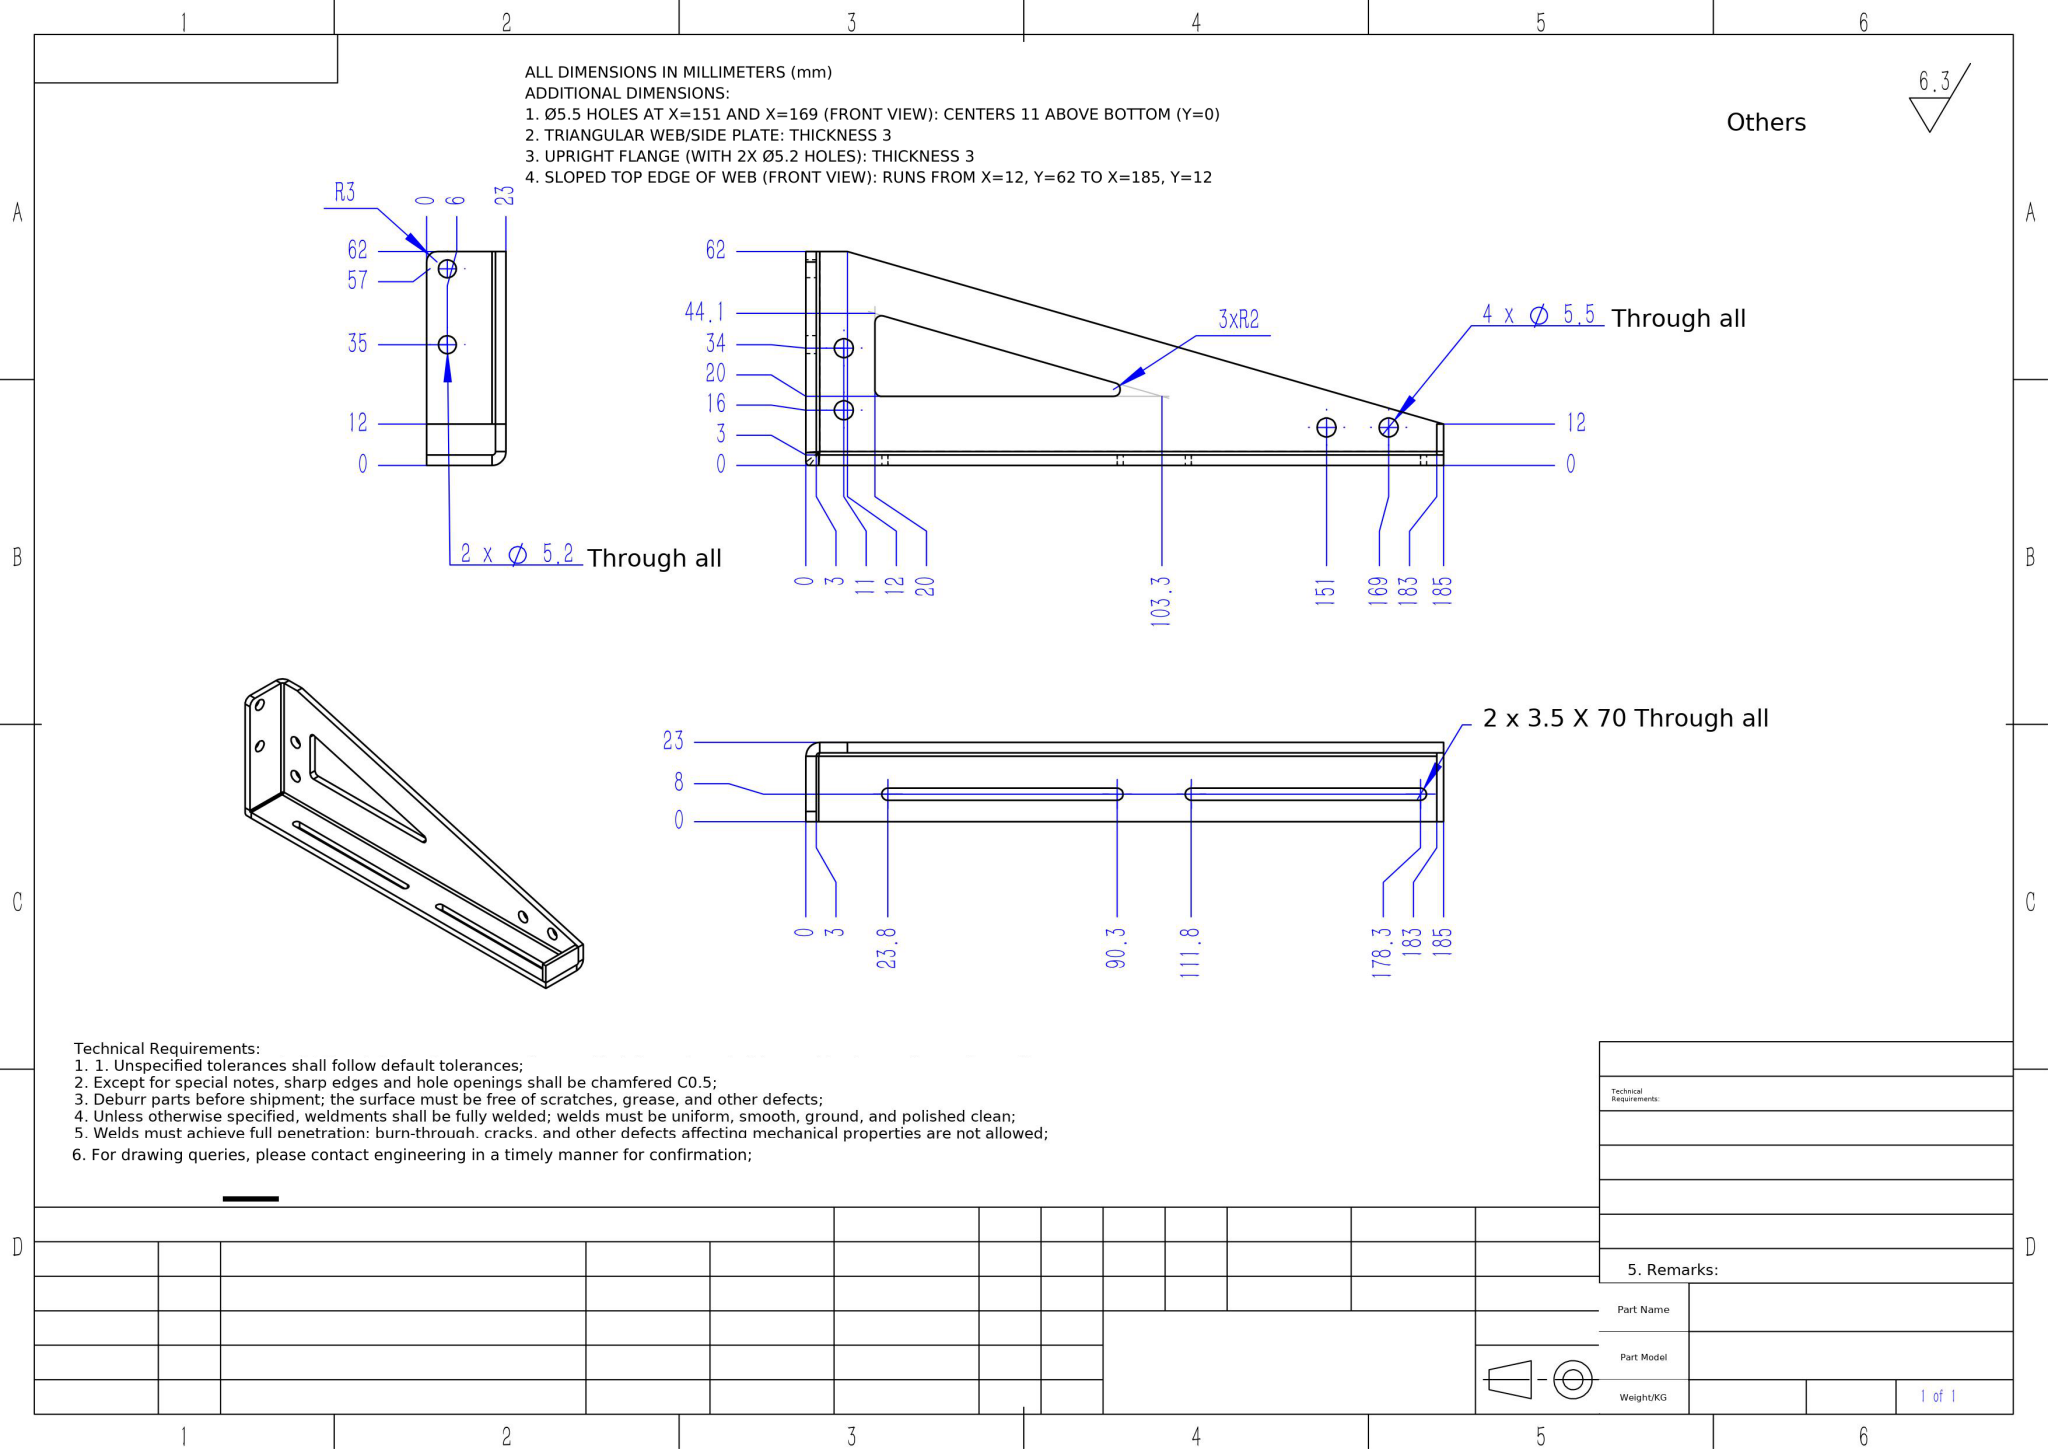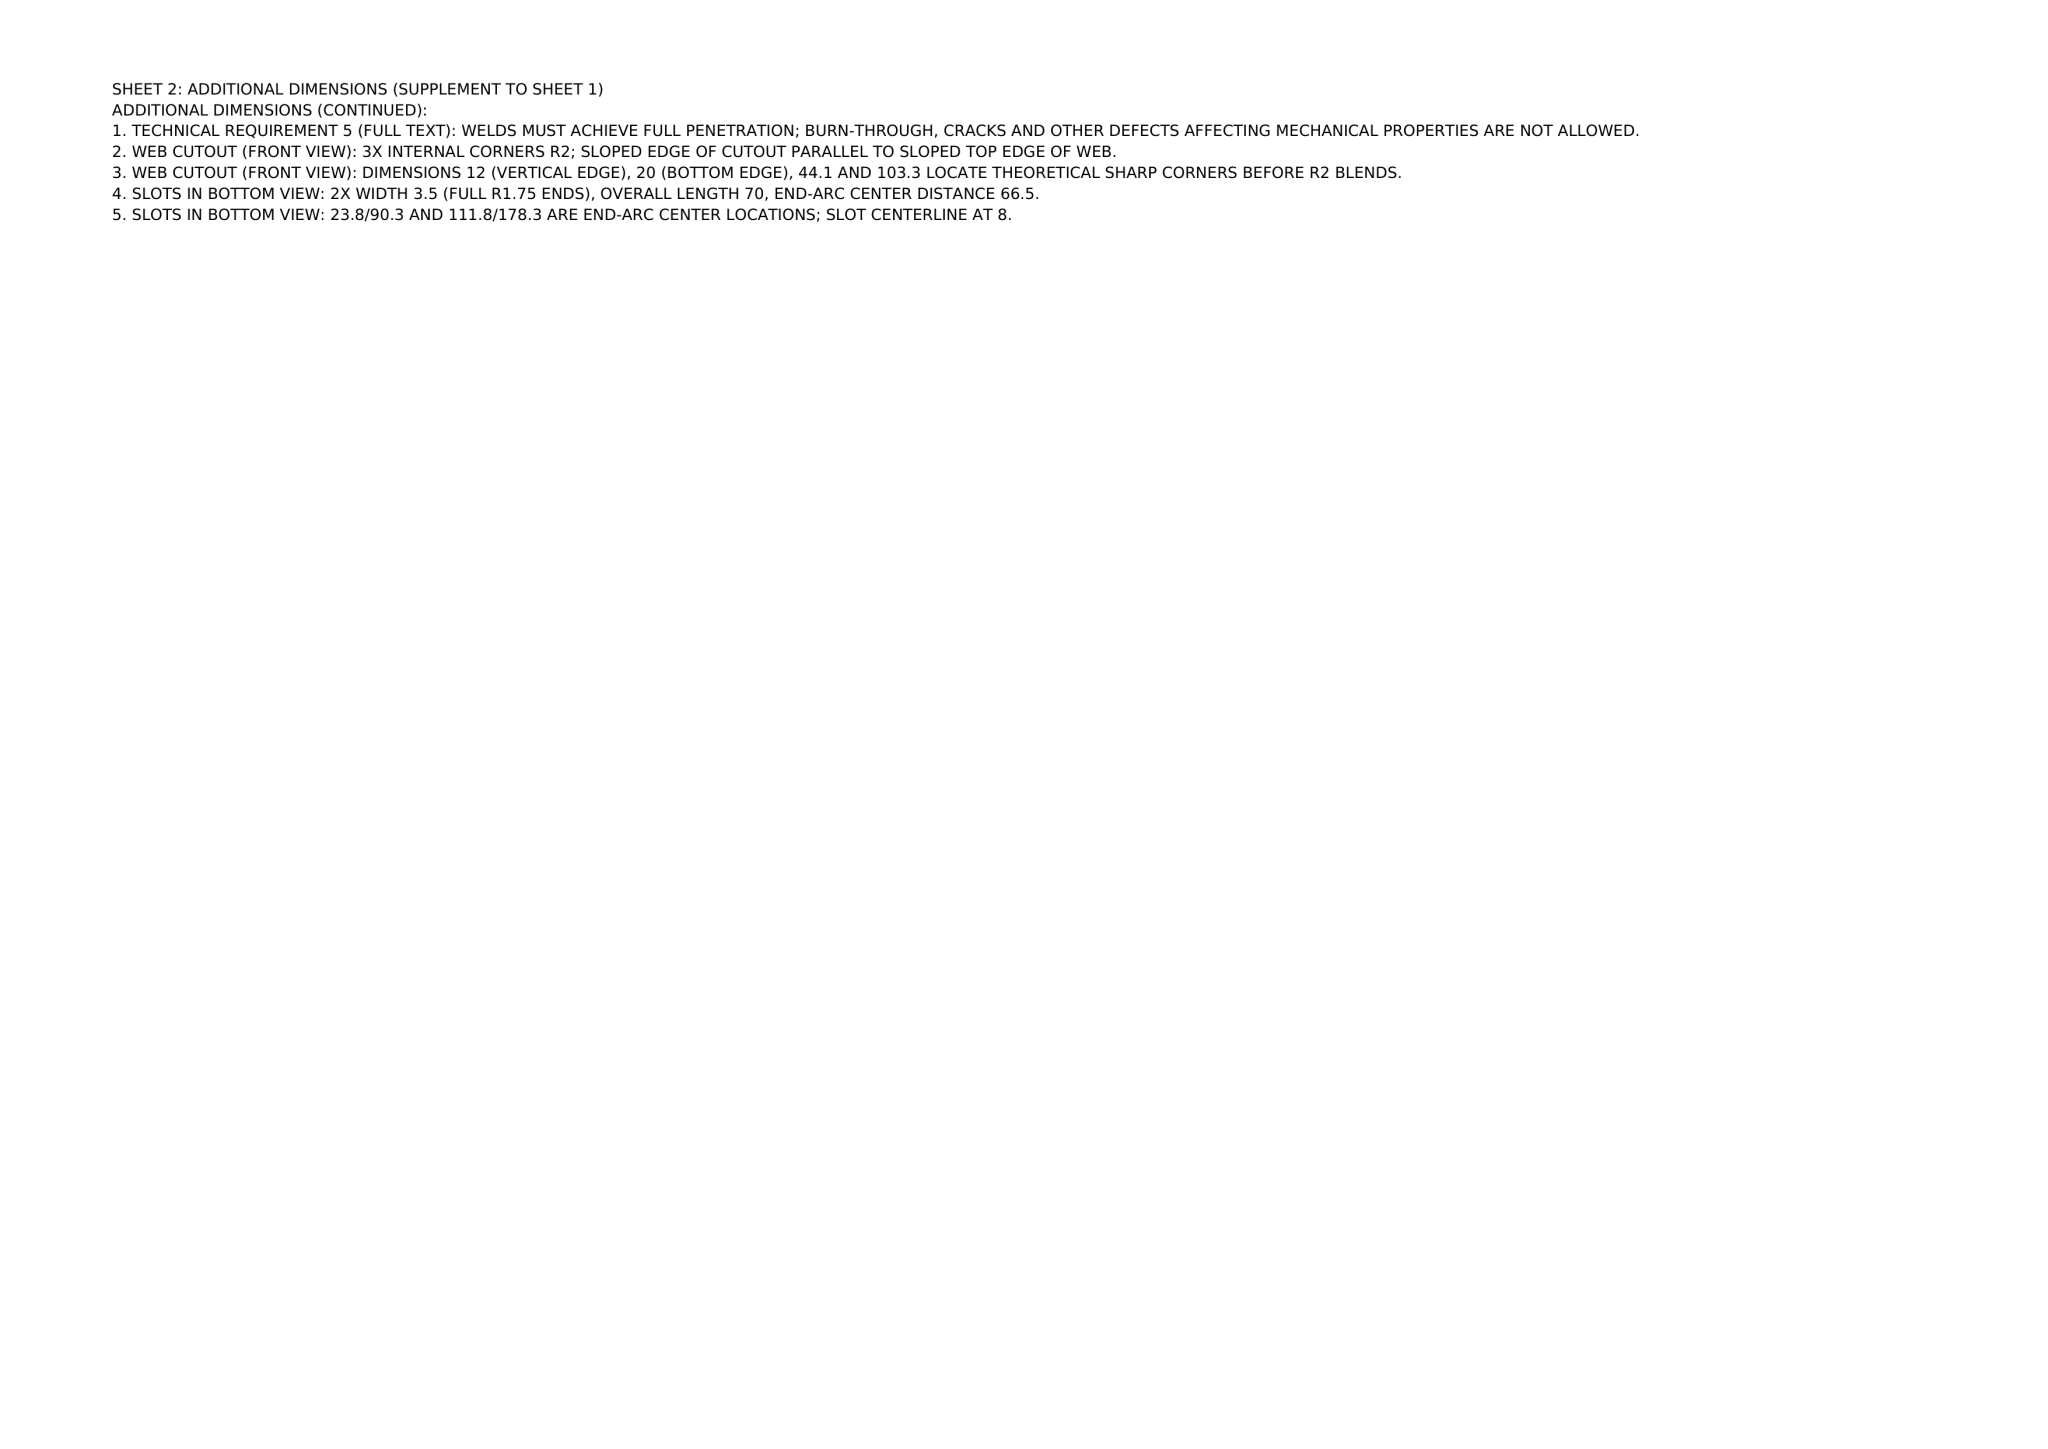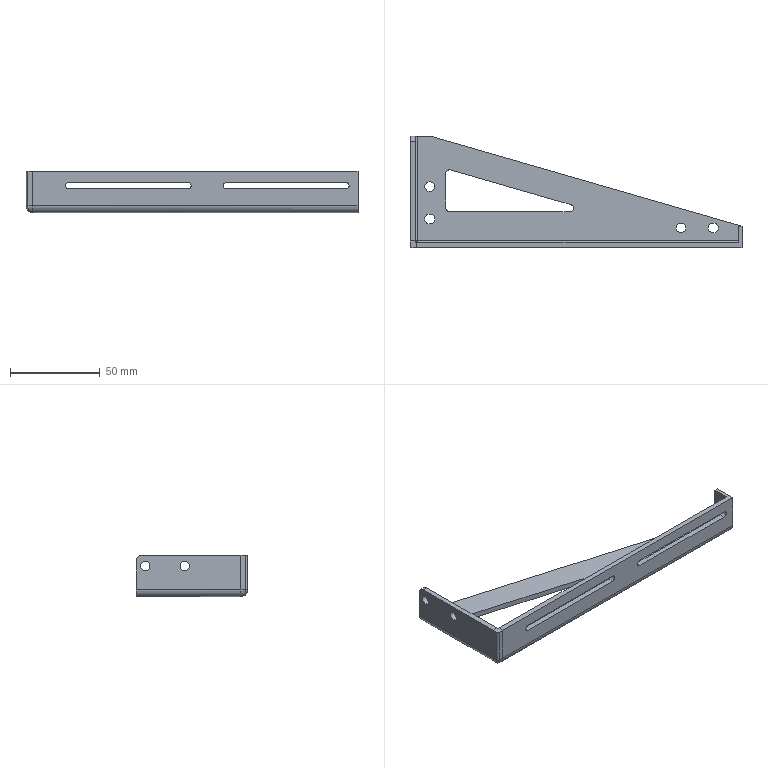Part | NX | mm | 1 solid | 57 faces | box 185 x 62 x 23 mm | volume 30835 mm3 | plane 27 | cylinder 25 | spline 5 | commonest cylinder face diameters 5.5 x8 5.2 x4 3.5 x4 4 x3 2 x3 8 x2 6 x1